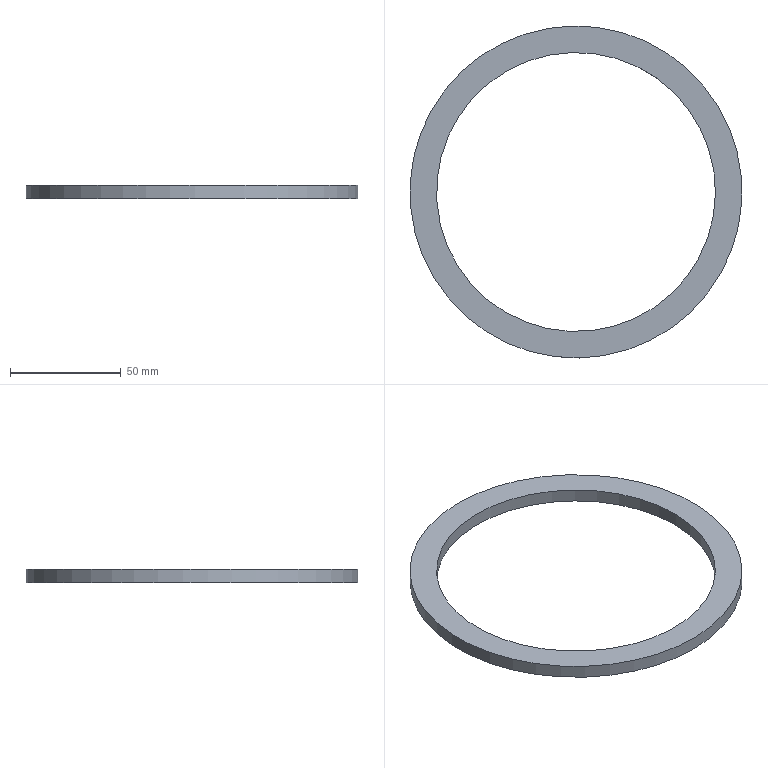Component | NX | CH3404-10 | 1 solid | 4 faces | box 150 x 150 x 6 mm | volume 31215 mm3 | cylinder 2 | plane 2 | commonest cylinder face diameters 150 x1 126 x1
STEP:
#1=CARTESIAN_POINT('',(0.,0.,0.));
#2=DIRECTION('',(0.,0.,1.));
#3=DIRECTION('',(1.,0.,0.));
#4=AXIS2_PLACEMENT_3D('',#1,#2,#3);
#5=CARTESIAN_POINT('',(-68.749,-28.623,-1536.3));
#6=VERTEX_POINT('',#5);
#7=CARTESIAN_POINT('',(0.5308,0.1057,-1536.3));
#8=DIRECTION('',(0.,0.,-1.));
#9=DIRECTION('',(-0.9237,-0.383,0.));
#10=AXIS2_PLACEMENT_3D('',#7,#8,#9);
#11=CIRCLE('',#10,75.);
#12=CARTESIAN_POINT('',(0.5308,0.1057,-1536.3));
#13=DIRECTION('',(0.,0.,1.));
#14=DIRECTION('',(0.9237,0.383,0.));
#15=AXIS2_PLACEMENT_3D('',#12,#13,#14);
#16=CYLINDRICAL_SURFACE('',#15,75.);
#17=CARTESIAN_POINT('',(9.425,0.));
#18=DIRECTION('',(-1.,0.));
#19=VECTOR('',#18,1.);
#20=LINE('',#17,#19);
#21=(GEOMETRIC_REPRESENTATION_CONTEXT(2)PARAMETRIC_REPRESENTATION_CONTEXT()REPRESENTATION_CONTEXT('',''));
#22=DEFINITIONAL_REPRESENTATION('',(#20),#21);
#23=PCURVE('',#16,#22);
#24=CARTESIAN_POINT('',(0.5308,0.1057,-1536.3));
#25=DIRECTION('',(0.,0.,-1.));
#26=DIRECTION('',(-0.9237,-0.383,0.));
#27=AXIS2_PLACEMENT_3D('',#24,#25,#26);
#28=PLANE('',#27);
#29=CARTESIAN_POINT('',(0.,0.));
#30=DIRECTION('',(1.,0.));
#31=AXIS2_PLACEMENT_2D('',#29,#30);
#32=CIRCLE('',#31,75.);
#33=(GEOMETRIC_REPRESENTATION_CONTEXT(2)PARAMETRIC_REPRESENTATION_CONTEXT()REPRESENTATION_CONTEXT('',''));
#34=DEFINITIONAL_REPRESENTATION('',(#32),#33);
#35=PCURVE('',#28,#34);
#36=SURFACE_CURVE('',#11,(#23,#35),.PCURVE_S1.);
#37=EDGE_CURVE('',#6,#6,#36,.T.);
#38=ORIENTED_EDGE('',*,*,#37,.F.);
#39=CARTESIAN_POINT('',(-68.749,-28.623,-1530.3));
#40=VERTEX_POINT('',#39);
#41=CARTESIAN_POINT('',(-68.749,-28.623,-1536.3));
#42=CARTESIAN_POINT('',(-68.749,-28.623,-1530.3));
#43=B_SPLINE_CURVE_WITH_KNOTS('',1,(#41,#42),.UNSPECIFIED.,.F.,.F.,(2,2),(0.,6.),.PIECEWISE_BEZIER_KNOTS.);
#44=CARTESIAN_POINT('',(9.425,0.));
#45=DIRECTION('',(0.,1.));
#46=VECTOR('',#45,1.);
#47=LINE('',#44,#46);
#48=(GEOMETRIC_REPRESENTATION_CONTEXT(2)PARAMETRIC_REPRESENTATION_CONTEXT()REPRESENTATION_CONTEXT('',''));
#49=DEFINITIONAL_REPRESENTATION('',(#47),#48);
#50=PCURVE('',#16,#49);
#51=CARTESIAN_POINT('',(3.142,0.));
#52=DIRECTION('',(0.,1.));
#53=VECTOR('',#52,1.);
#54=LINE('',#51,#53);
#55=(GEOMETRIC_REPRESENTATION_CONTEXT(2)PARAMETRIC_REPRESENTATION_CONTEXT()REPRESENTATION_CONTEXT('',''));
#56=DEFINITIONAL_REPRESENTATION('',(#54),#55);
#57=PCURVE('',#16,#56);
#58=SEAM_CURVE('',#43,(#50,#57),.PCURVE_S1.);
#59=EDGE_CURVE('',#6,#40,#58,.T.);
#60=ORIENTED_EDGE('',*,*,#59,.T.);
#61=CARTESIAN_POINT('',(0.5308,0.1057,-1530.3));
#62=DIRECTION('',(0.,0.,-1.));
#63=DIRECTION('',(-0.9237,-0.383,0.));
#64=AXIS2_PLACEMENT_3D('',#61,#62,#63);
#65=CIRCLE('',#64,75.);
#66=CARTESIAN_POINT('',(9.425,6.));
#67=DIRECTION('',(-1.,0.));
#68=VECTOR('',#67,1.);
#69=LINE('',#66,#68);
#70=(GEOMETRIC_REPRESENTATION_CONTEXT(2)PARAMETRIC_REPRESENTATION_CONTEXT()REPRESENTATION_CONTEXT('',''));
#71=DEFINITIONAL_REPRESENTATION('',(#69),#70);
#72=PCURVE('',#16,#71);
#73=CARTESIAN_POINT('',(0.5308,0.1057,-1530.3));
#74=DIRECTION('',(0.,0.,-1.));
#75=DIRECTION('',(-0.9237,-0.383,0.));
#76=AXIS2_PLACEMENT_3D('',#73,#74,#75);
#77=PLANE('',#76);
#78=CARTESIAN_POINT('',(0.,0.));
#79=DIRECTION('',(1.,0.));
#80=AXIS2_PLACEMENT_2D('',#78,#79);
#81=CIRCLE('',#80,75.);
#82=(GEOMETRIC_REPRESENTATION_CONTEXT(2)PARAMETRIC_REPRESENTATION_CONTEXT()REPRESENTATION_CONTEXT('',''));
#83=DEFINITIONAL_REPRESENTATION('',(#81),#82);
#84=PCURVE('',#77,#83);
#85=SURFACE_CURVE('',#65,(#72,#84),.PCURVE_S1.);
#86=EDGE_CURVE('',#40,#40,#85,.T.);
#87=ORIENTED_EDGE('',*,*,#86,.T.);
#88=ORIENTED_EDGE('',*,*,#59,.F.);
#89=EDGE_LOOP('',(#38,#60,#87,#88));
#90=FACE_BOUND('',#89,.T.);
#91=ADVANCED_FACE('',(#90),#16,.T.);
#92=CARTESIAN_POINT('',(-57.664,-24.026,-1536.3));
#93=VERTEX_POINT('',#92);
#94=CARTESIAN_POINT('',(0.5308,0.1057,-1536.3));
#95=DIRECTION('',(0.,0.,-1.));
#96=DIRECTION('',(-0.9237,-0.383,0.));
#97=AXIS2_PLACEMENT_3D('',#94,#95,#96);
#98=CIRCLE('',#97,63.);
#99=CARTESIAN_POINT('',(0.5308,0.1057,-1536.3));
#100=DIRECTION('',(0.,0.,1.));
#101=DIRECTION('',(0.9237,0.383,0.));
#102=AXIS2_PLACEMENT_3D('',#99,#100,#101);
#103=CYLINDRICAL_SURFACE('',#102,63.);
#104=CARTESIAN_POINT('',(9.425,0.));
#105=DIRECTION('',(-1.,0.));
#106=VECTOR('',#105,1.);
#107=LINE('',#104,#106);
#108=(GEOMETRIC_REPRESENTATION_CONTEXT(2)PARAMETRIC_REPRESENTATION_CONTEXT()REPRESENTATION_CONTEXT('',''));
#109=DEFINITIONAL_REPRESENTATION('',(#107),#108);
#110=PCURVE('',#103,#109);
#111=CARTESIAN_POINT('',(0.,0.));
#112=DIRECTION('',(1.,0.));
#113=AXIS2_PLACEMENT_2D('',#111,#112);
#114=CIRCLE('',#113,63.);
#115=(GEOMETRIC_REPRESENTATION_CONTEXT(2)PARAMETRIC_REPRESENTATION_CONTEXT()REPRESENTATION_CONTEXT('',''));
#116=DEFINITIONAL_REPRESENTATION('',(#114),#115);
#117=PCURVE('',#28,#116);
#118=SURFACE_CURVE('',#98,(#110,#117),.PCURVE_S1.);
#119=EDGE_CURVE('',#93,#93,#118,.T.);
#120=ORIENTED_EDGE('',*,*,#119,.F.);
#121=CARTESIAN_POINT('',(-57.664,-24.026,-1530.3));
#122=VERTEX_POINT('',#121);
#123=CARTESIAN_POINT('',(-57.664,-24.026,-1536.3));
#124=CARTESIAN_POINT('',(-57.664,-24.026,-1530.3));
#125=B_SPLINE_CURVE_WITH_KNOTS('',1,(#123,#124),.UNSPECIFIED.,.F.,.F.,(2,2),(0.,6.),.PIECEWISE_BEZIER_KNOTS.);
#126=CARTESIAN_POINT('',(9.425,0.));
#127=DIRECTION('',(0.,1.));
#128=VECTOR('',#127,1.);
#129=LINE('',#126,#128);
#130=(GEOMETRIC_REPRESENTATION_CONTEXT(2)PARAMETRIC_REPRESENTATION_CONTEXT()REPRESENTATION_CONTEXT('',''));
#131=DEFINITIONAL_REPRESENTATION('',(#129),#130);
#132=PCURVE('',#103,#131);
#133=CARTESIAN_POINT('',(3.142,0.));
#134=DIRECTION('',(0.,1.));
#135=VECTOR('',#134,1.);
#136=LINE('',#133,#135);
#137=(GEOMETRIC_REPRESENTATION_CONTEXT(2)PARAMETRIC_REPRESENTATION_CONTEXT()REPRESENTATION_CONTEXT('',''));
#138=DEFINITIONAL_REPRESENTATION('',(#136),#137);
#139=PCURVE('',#103,#138);
#140=SEAM_CURVE('',#125,(#132,#139),.PCURVE_S1.);
#141=EDGE_CURVE('',#93,#122,#140,.T.);
#142=ORIENTED_EDGE('',*,*,#141,.T.);
#143=CARTESIAN_POINT('',(0.5308,0.1057,-1530.3));
#144=DIRECTION('',(0.,0.,-1.));
#145=DIRECTION('',(-0.9237,-0.383,0.));
#146=AXIS2_PLACEMENT_3D('',#143,#144,#145);
#147=CIRCLE('',#146,63.);
#148=CARTESIAN_POINT('',(9.425,6.));
#149=DIRECTION('',(-1.,0.));
#150=VECTOR('',#149,1.);
#151=LINE('',#148,#150);
#152=(GEOMETRIC_REPRESENTATION_CONTEXT(2)PARAMETRIC_REPRESENTATION_CONTEXT()REPRESENTATION_CONTEXT('',''));
#153=DEFINITIONAL_REPRESENTATION('',(#151),#152);
#154=PCURVE('',#103,#153);
#155=CARTESIAN_POINT('',(0.,0.));
#156=DIRECTION('',(1.,0.));
#157=AXIS2_PLACEMENT_2D('',#155,#156);
#158=CIRCLE('',#157,63.);
#159=(GEOMETRIC_REPRESENTATION_CONTEXT(2)PARAMETRIC_REPRESENTATION_CONTEXT()REPRESENTATION_CONTEXT('',''));
#160=DEFINITIONAL_REPRESENTATION('',(#158),#159);
#161=PCURVE('',#77,#160);
#162=SURFACE_CURVE('',#147,(#154,#161),.PCURVE_S1.);
#163=EDGE_CURVE('',#122,#122,#162,.T.);
#164=ORIENTED_EDGE('',*,*,#163,.T.);
#165=ORIENTED_EDGE('',*,*,#141,.F.);
#166=EDGE_LOOP('',(#120,#142,#164,#165));
#167=FACE_BOUND('',#166,.F.);
#168=ADVANCED_FACE('',(#167),#103,.F.);
#169=ORIENTED_EDGE('',*,*,#37,.T.);
#170=EDGE_LOOP('',(#169));
#171=FACE_BOUND('',#170,.T.);
#172=ORIENTED_EDGE('',*,*,#119,.F.);
#173=EDGE_LOOP('',(#172));
#174=FACE_BOUND('',#173,.T.);
#175=ADVANCED_FACE('',(#171,#174),#28,.T.);
#176=ORIENTED_EDGE('',*,*,#86,.F.);
#177=EDGE_LOOP('',(#176));
#178=FACE_BOUND('',#177,.T.);
#179=ORIENTED_EDGE('',*,*,#163,.T.);
#180=EDGE_LOOP('',(#179));
#181=FACE_BOUND('',#180,.T.);
#182=ADVANCED_FACE('',(#178,#181),#77,.F.);
#183=CLOSED_SHELL('',(#91,#168,#175,#182));
#184=MANIFOLD_SOLID_BREP('',#183);
#185=(LENGTH_UNIT()NAMED_UNIT(*)SI_UNIT(.MILLI.,.METRE.));
#186=UNCERTAINTY_MEASURE_WITH_UNIT(LENGTH_MEASURE(0.00001),#185,'','');
#187=(NAMED_UNIT(*)PLANE_ANGLE_UNIT()SI_UNIT($,.RADIAN.));
#188=(NAMED_UNIT(*)SI_UNIT($,.STERADIAN.)SOLID_ANGLE_UNIT());
#189=(GEOMETRIC_REPRESENTATION_CONTEXT(3)GLOBAL_UNCERTAINTY_ASSIGNED_CONTEXT((#186))GLOBAL_UNIT_ASSIGNED_CONTEXT((#185,#187,#188))REPRESENTATION_CONTEXT('',''));
#190=ADVANCED_BREP_SHAPE_REPRESENTATION('',(#4,#184),#189);